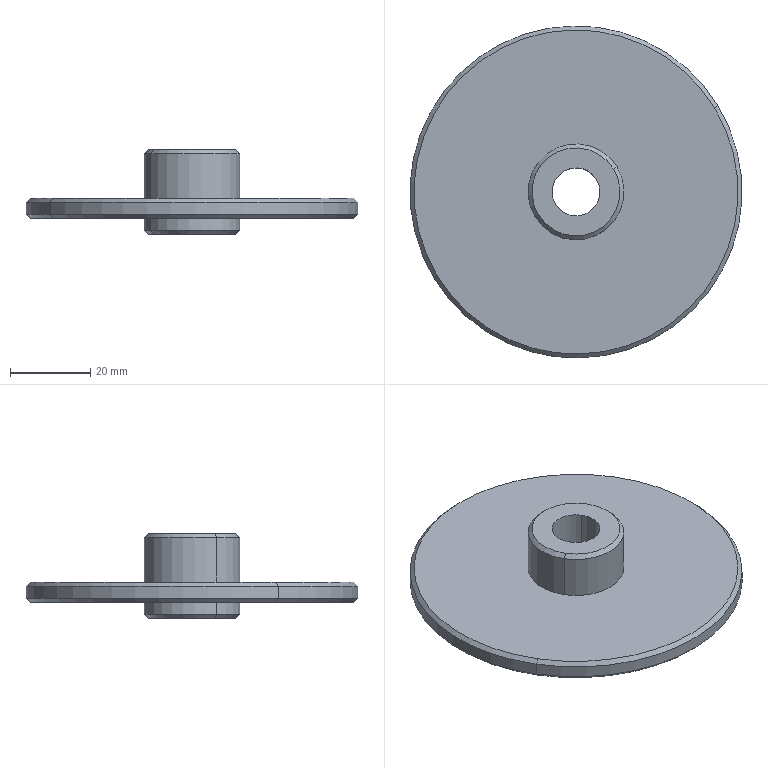Component | SolidWorks | TAR-02-033PaperStopWheel-1 | 1 solid | 20 faces | box 83 x 83 x 21 mm | volume 31584 mm3 | cone 8 | cylinder 8 | plane 4 | commonest cylinder face diameters 24 x4 12 x2 83 x2
build123d program:
from build123d import *

# Parameters (mm, degrees)
SKETCH1_R           = 12
BOSS_EXTRUDE1_DEPTH = 4
SKETCH2_R           = 41.5
BOSS_EXTRUDE2_DEPTH = 5
SKETCH3_R           = 12
BOSS_EXTRUDE3_DEPTH = 12
SKETCH4_R           = 6
CUT_EXTRUDE1_DEPTH  = 99
CHAMFER1_SIZE       = 1


with BuildPart() as part:
    # Sketch1 → Boss-Extrude1 (new body)
    with BuildSketch(Plane.XY):
        Circle(SKETCH1_R)
    extrude(amount=BOSS_EXTRUDE1_DEPTH)

    # Sketch2 → Boss-Extrude2 (add)
    with BuildSketch(Plane.XY.offset(4)):
        Circle(SKETCH2_R)
    extrude(amount=BOSS_EXTRUDE2_DEPTH)

    # Sketch3 → Boss-Extrude3 (add)
    with BuildSketch(Plane.XY.offset(9)):
        Circle(SKETCH3_R)
    extrude(amount=BOSS_EXTRUDE3_DEPTH)

    # Sketch4 → Cut-Extrude1 (cut)
    with BuildSketch(Plane.XY.offset(21)):
        Circle(SKETCH4_R)
    extrude(amount=-CUT_EXTRUDE1_DEPTH, mode=Mode.SUBTRACT)

    # Chamfer1
    chamfer1_edges = [part.edges().sort_by_distance(p)[0] for p in [
        (-12, 0, 21),
        (-12, 0, 0),
        (-41.5, 0, 4),
        (-41.5, 0, 9),
    ]]
    chamfer(chamfer1_edges, length=CHAMFER1_SIZE)


solid = part.part

# Placed as in the assembly
solid = solid.moved(Location((-115.391, 9.288, -85.4), (0, 0, 0)))
STEP:
#1=COLOUR_RGB('',0.7922,0.8196,0.9333);
#2=FILL_AREA_STYLE_COLOUR('',#1);
#3=FILL_AREA_STYLE('',(#2));
#4=SURFACE_STYLE_FILL_AREA(#3);
#5=SURFACE_SIDE_STYLE('',(#4));
#6=SURFACE_STYLE_USAGE(.BOTH.,#5);
#7=PRESENTATION_STYLE_ASSIGNMENT((#6));
#8=CARTESIAN_POINT('',(-4.173,0.5905,-2.535));
#9=VERTEX_POINT('',#8);
#10=CARTESIAN_POINT('',(-4.913,0.1408,-2.535));
#11=VERTEX_POINT('',#10);
#12=CARTESIAN_POINT('',(-4.543,0.3657,-2.535));
#13=DIRECTION('',(0.,0.,1.));
#14=DIRECTION('',(0.8546,0.5192,0.));
#15=AXIS2_PLACEMENT_3D('',#12,#13,#14);
#16=CIRCLE('',#15,0.4331);
#17=EDGE_CURVE('',#9,#11,#16,.T.);
#18=ORIENTED_EDGE('',*,*,#17,.F.);
#19=CARTESIAN_POINT('',(-4.139,0.611,-2.575));
#20=VERTEX_POINT('',#19);
#21=CARTESIAN_POINT('',(-4.173,0.5905,-2.535));
#22=DIRECTION('',(0.6043,0.3671,-0.7071));
#23=VECTOR('',#22,39.37);
#24=LINE('',#21,#23);
#25=EDGE_CURVE('',#9,#20,#24,.T.);
#26=ORIENTED_EDGE('',*,*,#25,.T.);
#27=CARTESIAN_POINT('',(-4.947,0.1204,-2.575));
#28=VERTEX_POINT('',#27);
#29=CARTESIAN_POINT('',(-4.543,0.3657,-2.575));
#30=DIRECTION('',(0.,0.,-1.));
#31=DIRECTION('',(0.8546,0.5192,0.));
#32=AXIS2_PLACEMENT_3D('',#29,#30,#31);
#33=CIRCLE('',#32,0.4724);
#34=EDGE_CURVE('',#28,#20,#33,.T.);
#35=ORIENTED_EDGE('',*,*,#34,.F.);
#36=CARTESIAN_POINT('',(-4.913,0.1408,-2.535));
#37=DIRECTION('',(-0.6043,-0.3671,-0.7071));
#38=VECTOR('',#37,39.37);
#39=LINE('',#36,#38);
#40=EDGE_CURVE('',#11,#28,#39,.T.);
#41=ORIENTED_EDGE('',*,*,#40,.F.);
#42=EDGE_LOOP('',(#18,#26,#35,#41));
#43=FACE_OUTER_BOUND('',#42,.T.);
#44=CARTESIAN_POINT('',(-4.543,0.3657,-2.535));
#45=DIRECTION('',(0.,0.,-1.));
#46=DIRECTION('',(-0.8546,-0.5192,0.));
#47=AXIS2_PLACEMENT_3D('',#44,#45,#46);
#48=CONICAL_SURFACE('',#47,0.4331,0.7854);
#49=ADVANCED_FACE('',(#43),#48,.T.);
#50=CARTESIAN_POINT('',(-4.913,0.1408,-3.362));
#51=VERTEX_POINT('',#50);
#52=CARTESIAN_POINT('',(-4.173,0.5905,-3.362));
#53=VERTEX_POINT('',#52);
#54=CARTESIAN_POINT('',(-4.543,0.3657,-3.362));
#55=DIRECTION('',(0.,0.,-1.));
#56=DIRECTION('',(0.8546,0.5192,0.));
#57=AXIS2_PLACEMENT_3D('',#54,#55,#56);
#58=CIRCLE('',#57,0.4331);
#59=EDGE_CURVE('',#51,#53,#58,.T.);
#60=ORIENTED_EDGE('',*,*,#59,.F.);
#61=CARTESIAN_POINT('',(-4.947,0.1204,-3.323));
#62=VERTEX_POINT('',#61);
#63=CARTESIAN_POINT('',(-4.947,0.1204,-3.323));
#64=DIRECTION('',(-0.6043,-0.3671,0.7071));
#65=VECTOR('',#64,39.37);
#66=LINE('',#63,#65);
#67=EDGE_CURVE('',#51,#62,#66,.T.);
#68=ORIENTED_EDGE('',*,*,#67,.T.);
#69=CARTESIAN_POINT('',(-4.139,0.611,-3.323));
#70=VERTEX_POINT('',#69);
#71=CARTESIAN_POINT('',(-4.543,0.3657,-3.323));
#72=DIRECTION('',(0.,0.,1.));
#73=DIRECTION('',(0.8546,0.5192,0.));
#74=AXIS2_PLACEMENT_3D('',#71,#72,#73);
#75=CIRCLE('',#74,0.4724);
#76=EDGE_CURVE('',#70,#62,#75,.T.);
#77=ORIENTED_EDGE('',*,*,#76,.F.);
#78=CARTESIAN_POINT('',(-4.139,0.611,-3.323));
#79=DIRECTION('',(0.6043,0.3671,0.7071));
#80=VECTOR('',#79,39.37);
#81=LINE('',#78,#80);
#82=EDGE_CURVE('',#53,#70,#81,.T.);
#83=ORIENTED_EDGE('',*,*,#82,.F.);
#84=EDGE_LOOP('',(#60,#68,#77,#83));
#85=FACE_OUTER_BOUND('',#84,.T.);
#86=CARTESIAN_POINT('',(-4.543,0.3657,-3.323));
#87=DIRECTION('',(0.,0.,1.));
#88=DIRECTION('',(0.8546,0.5192,0.));
#89=AXIS2_PLACEMENT_3D('',#86,#87,#88);
#90=CONICAL_SURFACE('',#89,0.4724,0.7854);
#91=ADVANCED_FACE('',(#85),#90,.T.);
#92=CARTESIAN_POINT('',(-3.18,1.194,-3.008));
#93=VERTEX_POINT('',#92);
#94=CARTESIAN_POINT('',(-5.906,-0.4622,-3.008));
#95=VERTEX_POINT('',#94);
#96=CARTESIAN_POINT('',(-4.543,0.3657,-3.008));
#97=DIRECTION('',(0.,0.,1.));
#98=DIRECTION('',(0.8546,0.5192,0.));
#99=AXIS2_PLACEMENT_3D('',#96,#97,#98);
#100=CIRCLE('',#99,1.594);
#101=EDGE_CURVE('',#93,#95,#100,.T.);
#102=ORIENTED_EDGE('',*,*,#101,.F.);
#103=CARTESIAN_POINT('',(-3.147,1.214,-3.047));
#104=VERTEX_POINT('',#103);
#105=CARTESIAN_POINT('',(-3.18,1.194,-3.008));
#106=DIRECTION('',(0.6043,0.3671,-0.7071));
#107=VECTOR('',#106,39.37);
#108=LINE('',#105,#107);
#109=EDGE_CURVE('',#93,#104,#108,.T.);
#110=ORIENTED_EDGE('',*,*,#109,.T.);
#111=CARTESIAN_POINT('',(-5.939,-0.4827,-3.047));
#112=VERTEX_POINT('',#111);
#113=CARTESIAN_POINT('',(-4.543,0.3657,-3.047));
#114=DIRECTION('',(0.,0.,-1.));
#115=DIRECTION('',(0.8546,0.5192,0.));
#116=AXIS2_PLACEMENT_3D('',#113,#114,#115);
#117=CIRCLE('',#116,1.634);
#118=EDGE_CURVE('',#112,#104,#117,.T.);
#119=ORIENTED_EDGE('',*,*,#118,.F.);
#120=CARTESIAN_POINT('',(-5.906,-0.4622,-3.008));
#121=DIRECTION('',(-0.6043,-0.3671,-0.7071));
#122=VECTOR('',#121,39.37);
#123=LINE('',#120,#122);
#124=EDGE_CURVE('',#95,#112,#123,.T.);
#125=ORIENTED_EDGE('',*,*,#124,.F.);
#126=EDGE_LOOP('',(#102,#110,#119,#125));
#127=FACE_OUTER_BOUND('',#126,.T.);
#128=CARTESIAN_POINT('',(-4.543,0.3657,-3.008));
#129=DIRECTION('',(0.,0.,-1.));
#130=DIRECTION('',(-0.8546,-0.5192,0.));
#131=AXIS2_PLACEMENT_3D('',#128,#129,#130);
#132=CONICAL_SURFACE('',#131,1.594,0.7854);
#133=ADVANCED_FACE('',(#127),#132,.T.);
#134=CARTESIAN_POINT('',(-5.906,-0.4622,-3.205));
#135=VERTEX_POINT('',#134);
#136=CARTESIAN_POINT('',(-3.18,1.194,-3.205));
#137=VERTEX_POINT('',#136);
#138=CARTESIAN_POINT('',(-4.543,0.3657,-3.205));
#139=DIRECTION('',(0.,0.,-1.));
#140=DIRECTION('',(0.8546,0.5192,0.));
#141=AXIS2_PLACEMENT_3D('',#138,#139,#140);
#142=CIRCLE('',#141,1.594);
#143=EDGE_CURVE('',#135,#137,#142,.T.);
#144=ORIENTED_EDGE('',*,*,#143,.F.);
#145=CARTESIAN_POINT('',(-5.939,-0.4827,-3.165));
#146=VERTEX_POINT('',#145);
#147=CARTESIAN_POINT('',(-5.939,-0.4827,-3.165));
#148=DIRECTION('',(-0.6043,-0.3671,0.7071));
#149=VECTOR('',#148,39.37);
#150=LINE('',#147,#149);
#151=EDGE_CURVE('',#135,#146,#150,.T.);
#152=ORIENTED_EDGE('',*,*,#151,.T.);
#153=CARTESIAN_POINT('',(-3.147,1.214,-3.165));
#154=VERTEX_POINT('',#153);
#155=CARTESIAN_POINT('',(-4.543,0.3657,-3.165));
#156=DIRECTION('',(0.,0.,1.));
#157=DIRECTION('',(0.8546,0.5192,0.));
#158=AXIS2_PLACEMENT_3D('',#155,#156,#157);
#159=CIRCLE('',#158,1.634);
#160=EDGE_CURVE('',#154,#146,#159,.T.);
#161=ORIENTED_EDGE('',*,*,#160,.F.);
#162=CARTESIAN_POINT('',(-3.147,1.214,-3.165));
#163=DIRECTION('',(0.6043,0.3671,0.7071));
#164=VECTOR('',#163,39.37);
#165=LINE('',#162,#164);
#166=EDGE_CURVE('',#137,#154,#165,.T.);
#167=ORIENTED_EDGE('',*,*,#166,.F.);
#168=EDGE_LOOP('',(#144,#152,#161,#167));
#169=FACE_OUTER_BOUND('',#168,.T.);
#170=CARTESIAN_POINT('',(-4.543,0.3657,-3.165));
#171=DIRECTION('',(0.,0.,1.));
#172=DIRECTION('',(0.8546,0.5192,0.));
#173=AXIS2_PLACEMENT_3D('',#170,#171,#172);
#174=CONICAL_SURFACE('',#173,1.634,0.7854);
#175=ADVANCED_FACE('',(#169),#174,.T.);
#176=CARTESIAN_POINT('',(-4.745,0.243,-3.362));
#177=VERTEX_POINT('',#176);
#178=CARTESIAN_POINT('',(-4.341,0.4883,-3.362));
#179=VERTEX_POINT('',#178);
#180=CARTESIAN_POINT('',(-4.543,0.3657,-3.362));
#181=DIRECTION('',(0.,0.,1.));
#182=DIRECTION('',(0.8546,0.5192,0.));
#183=AXIS2_PLACEMENT_3D('',#180,#181,#182);
#184=CIRCLE('',#183,0.2362);
#185=EDGE_CURVE('',#177,#179,#184,.T.);
#186=ORIENTED_EDGE('',*,*,#185,.F.);
#187=CARTESIAN_POINT('',(-4.745,0.243,-2.535));
#188=VERTEX_POINT('',#187);
#189=CARTESIAN_POINT('',(-4.745,0.243,-6.433));
#190=DIRECTION('',(0.,0.,1.));
#191=VECTOR('',#190,39.37);
#192=LINE('',#189,#191);
#193=EDGE_CURVE('',#177,#188,#192,.T.);
#194=ORIENTED_EDGE('',*,*,#193,.T.);
#195=CARTESIAN_POINT('',(-4.341,0.4883,-2.535));
#196=VERTEX_POINT('',#195);
#197=CARTESIAN_POINT('',(-4.543,0.3657,-2.535));
#198=DIRECTION('',(0.,0.,1.));
#199=DIRECTION('',(0.8546,0.5192,0.));
#200=AXIS2_PLACEMENT_3D('',#197,#198,#199);
#201=CIRCLE('',#200,0.2362);
#202=EDGE_CURVE('',#188,#196,#201,.T.);
#203=ORIENTED_EDGE('',*,*,#202,.T.);
#204=CARTESIAN_POINT('',(-4.341,0.4883,-6.433));
#205=DIRECTION('',(0.,0.,1.));
#206=VECTOR('',#205,39.37);
#207=LINE('',#204,#206);
#208=EDGE_CURVE('',#179,#196,#207,.T.);
#209=ORIENTED_EDGE('',*,*,#208,.F.);
#210=EDGE_LOOP('',(#186,#194,#203,#209));
#211=FACE_OUTER_BOUND('',#210,.T.);
#212=CARTESIAN_POINT('',(-4.543,0.3657,-6.433));
#213=DIRECTION('',(0.,0.,1.));
#214=DIRECTION('',(0.8546,0.5192,0.));
#215=AXIS2_PLACEMENT_3D('',#212,#213,#214);
#216=CYLINDRICAL_SURFACE('',#215,0.2362);
#217=ADVANCED_FACE('',(#211),#216,.F.);
#218=ORIENTED_EDGE('',*,*,#34,.T.);
#219=CARTESIAN_POINT('',(-4.139,0.611,-3.008));
#220=VERTEX_POINT('',#219);
#221=CARTESIAN_POINT('',(-4.139,0.611,-2.535));
#222=DIRECTION('',(0.,0.,-1.));
#223=VECTOR('',#222,39.37);
#224=LINE('',#221,#223);
#225=EDGE_CURVE('',#20,#220,#224,.T.);
#226=ORIENTED_EDGE('',*,*,#225,.T.);
#227=CARTESIAN_POINT('',(-4.947,0.1204,-3.008));
#228=VERTEX_POINT('',#227);
#229=CARTESIAN_POINT('',(-4.543,0.3657,-3.008));
#230=DIRECTION('',(0.,0.,1.));
#231=DIRECTION('',(0.8546,0.5192,0.));
#232=AXIS2_PLACEMENT_3D('',#229,#230,#231);
#233=CIRCLE('',#232,0.4724);
#234=EDGE_CURVE('',#220,#228,#233,.T.);
#235=ORIENTED_EDGE('',*,*,#234,.T.);
#236=CARTESIAN_POINT('',(-4.947,0.1204,-2.535));
#237=DIRECTION('',(0.,0.,-1.));
#238=VECTOR('',#237,39.37);
#239=LINE('',#236,#238);
#240=EDGE_CURVE('',#28,#228,#239,.T.);
#241=ORIENTED_EDGE('',*,*,#240,.F.);
#242=EDGE_LOOP('',(#218,#226,#235,#241));
#243=FACE_OUTER_BOUND('',#242,.T.);
#244=CARTESIAN_POINT('',(-4.543,0.3657,-2.535));
#245=DIRECTION('',(0.,0.,-1.));
#246=DIRECTION('',(-0.8546,-0.5192,0.));
#247=AXIS2_PLACEMENT_3D('',#244,#245,#246);
#248=CYLINDRICAL_SURFACE('',#247,0.4724);
#249=ADVANCED_FACE('',(#243),#248,.T.);
#250=ORIENTED_EDGE('',*,*,#118,.T.);
#251=CARTESIAN_POINT('',(-3.147,1.214,-3.008));
#252=DIRECTION('',(0.,0.,-1.));
#253=VECTOR('',#252,39.37);
#254=LINE('',#251,#253);
#255=EDGE_CURVE('',#104,#154,#254,.T.);
#256=ORIENTED_EDGE('',*,*,#255,.T.);
#257=ORIENTED_EDGE('',*,*,#160,.T.);
#258=CARTESIAN_POINT('',(-5.939,-0.4827,-3.008));
#259=DIRECTION('',(0.,0.,-1.));
#260=VECTOR('',#259,39.37);
#261=LINE('',#258,#260);
#262=EDGE_CURVE('',#112,#146,#261,.T.);
#263=ORIENTED_EDGE('',*,*,#262,.F.);
#264=EDGE_LOOP('',(#250,#256,#257,#263));
#265=FACE_OUTER_BOUND('',#264,.T.);
#266=CARTESIAN_POINT('',(-4.543,0.3657,-3.008));
#267=DIRECTION('',(0.,0.,-1.));
#268=DIRECTION('',(-0.8546,-0.5192,0.));
#269=AXIS2_PLACEMENT_3D('',#266,#267,#268);
#270=CYLINDRICAL_SURFACE('',#269,1.634);
#271=ADVANCED_FACE('',(#265),#270,.T.);
#272=CARTESIAN_POINT('',(-4.139,0.611,-3.205));
#273=VERTEX_POINT('',#272);
#274=CARTESIAN_POINT('',(-4.947,0.1204,-3.205));
#275=VERTEX_POINT('',#274);
#276=CARTESIAN_POINT('',(-4.543,0.3657,-3.205));
#277=DIRECTION('',(0.,0.,1.));
#278=DIRECTION('',(0.8546,0.5192,0.));
#279=AXIS2_PLACEMENT_3D('',#276,#277,#278);
#280=CIRCLE('',#279,0.4724);
#281=EDGE_CURVE('',#273,#275,#280,.T.);
#282=ORIENTED_EDGE('',*,*,#281,.F.);
#283=CARTESIAN_POINT('',(-4.139,0.611,-3.205));
#284=DIRECTION('',(0.,0.,-1.));
#285=VECTOR('',#284,39.37);
#286=LINE('',#283,#285);
#287=EDGE_CURVE('',#273,#70,#286,.T.);
#288=ORIENTED_EDGE('',*,*,#287,.T.);
#289=ORIENTED_EDGE('',*,*,#76,.T.);
#290=CARTESIAN_POINT('',(-4.947,0.1204,-3.205));
#291=DIRECTION('',(0.,0.,-1.));
#292=VECTOR('',#291,39.37);
#293=LINE('',#290,#292);
#294=EDGE_CURVE('',#275,#62,#293,.T.);
#295=ORIENTED_EDGE('',*,*,#294,.F.);
#296=EDGE_LOOP('',(#282,#288,#289,#295));
#297=FACE_OUTER_BOUND('',#296,.T.);
#298=CARTESIAN_POINT('',(-4.543,0.3657,-3.205));
#299=DIRECTION('',(0.,0.,-1.));
#300=DIRECTION('',(-0.8546,-0.5192,0.));
#301=AXIS2_PLACEMENT_3D('',#298,#299,#300);
#302=CYLINDRICAL_SURFACE('',#301,0.4724);
#303=ADVANCED_FACE('',(#297),#302,.T.);
#304=ORIENTED_EDGE('',*,*,#287,.F.);
#305=CARTESIAN_POINT('',(-4.543,0.3657,-3.205));
#306=DIRECTION('',(0.,0.,1.));
#307=DIRECTION('',(0.8546,0.5192,0.));
#308=AXIS2_PLACEMENT_3D('',#305,#306,#307);
#309=CIRCLE('',#308,0.4724);
#310=EDGE_CURVE('',#275,#273,#309,.T.);
#311=ORIENTED_EDGE('',*,*,#310,.F.);
#312=ORIENTED_EDGE('',*,*,#294,.T.);
#313=CARTESIAN_POINT('',(-4.543,0.3657,-3.323));
#314=DIRECTION('',(0.,0.,1.));
#315=DIRECTION('',(0.8546,0.5192,0.));
#316=AXIS2_PLACEMENT_3D('',#313,#314,#315);
#317=CIRCLE('',#316,0.4724);
#318=EDGE_CURVE('',#62,#70,#317,.T.);
#319=ORIENTED_EDGE('',*,*,#318,.T.);
#320=EDGE_LOOP('',(#304,#311,#312,#319));
#321=FACE_OUTER_BOUND('',#320,.T.);
#322=CARTESIAN_POINT('',(-4.543,0.3657,-3.205));
#323=DIRECTION('',(0.,0.,-1.));
#324=DIRECTION('',(-0.8546,-0.5192,0.));
#325=AXIS2_PLACEMENT_3D('',#322,#323,#324);
#326=CYLINDRICAL_SURFACE('',#325,0.4724);
#327=ADVANCED_FACE('',(#321),#326,.T.);
#328=CARTESIAN_POINT('',(-4.543,0.3657,-3.362));
#329=DIRECTION('',(0.,0.,-1.));
#330=DIRECTION('',(0.8546,0.5192,0.));
#331=AXIS2_PLACEMENT_3D('',#328,#329,#330);
#332=CIRCLE('',#331,0.4331);
#333=EDGE_CURVE('',#53,#51,#332,.T.);
#334=ORIENTED_EDGE('',*,*,#333,.T.);
#335=ORIENTED_EDGE('',*,*,#59,.T.);
#336=EDGE_LOOP('',(#334,#335));
#337=FACE_OUTER_BOUND('',#336,.T.);
#338=CARTESIAN_POINT('',(-4.543,0.3657,-3.362));
#339=DIRECTION('',(0.,0.,1.));
#340=DIRECTION('',(0.8546,0.5192,0.));
#341=AXIS2_PLACEMENT_3D('',#338,#339,#340);
#342=CIRCLE('',#341,0.2362);
#343=EDGE_CURVE('',#179,#177,#342,.T.);
#344=ORIENTED_EDGE('',*,*,#343,.T.);
#345=ORIENTED_EDGE('',*,*,#185,.T.);
#346=EDGE_LOOP('',(#344,#345));
#347=FACE_BOUND('',#346,.T.);
#348=CARTESIAN_POINT('',(-4.543,0.3657,-3.362));
#349=DIRECTION('',(0.,0.,1.));
#350=DIRECTION('',(0.8546,0.5192,0.));
#351=AXIS2_PLACEMENT_3D('',#348,#349,#350);
#352=PLANE('',#351);
#353=ADVANCED_FACE('',(#337,#347),#352,.F.);
#354=ORIENTED_EDGE('',*,*,#255,.F.);
#355=CARTESIAN_POINT('',(-4.543,0.3657,-3.047));
#356=DIRECTION('',(0.,0.,-1.));
#357=DIRECTION('',(0.8546,0.5192,0.));
#358=AXIS2_PLACEMENT_3D('',#355,#356,#357);
#359=CIRCLE('',#358,1.634);
#360=EDGE_CURVE('',#104,#112,#359,.T.);
#361=ORIENTED_EDGE('',*,*,#360,.T.);
#362=ORIENTED_EDGE('',*,*,#262,.T.);
#363=CARTESIAN_POINT('',(-4.543,0.3657,-3.165));
#364=DIRECTION('',(0.,0.,1.));
#365=DIRECTION('',(0.8546,0.5192,0.));
#366=AXIS2_PLACEMENT_3D('',#363,#364,#365);
#367=CIRCLE('',#366,1.634);
#368=EDGE_CURVE('',#146,#154,#367,.T.);
#369=ORIENTED_EDGE('',*,*,#368,.T.);
#370=EDGE_LOOP('',(#354,#361,#362,#369));
#371=FACE_OUTER_BOUND('',#370,.T.);
#372=CARTESIAN_POINT('',(-4.543,0.3657,-3.008));
#373=DIRECTION('',(0.,0.,-1.));
#374=DIRECTION('',(-0.8546,-0.5192,0.));
#375=AXIS2_PLACEMENT_3D('',#372,#373,#374);
#376=CYLINDRICAL_SURFACE('',#375,1.634);
#377=ADVANCED_FACE('',(#371),#376,.T.);
#378=CARTESIAN_POINT('',(-4.543,0.3657,-3.008));
#379=DIRECTION('',(0.,0.,1.));
#380=DIRECTION('',(0.8546,0.5192,0.));
#381=AXIS2_PLACEMENT_3D('',#378,#379,#380);
#382=CIRCLE('',#381,1.594);
#383=EDGE_CURVE('',#95,#93,#382,.T.);
#384=ORIENTED_EDGE('',*,*,#383,.T.);
#385=ORIENTED_EDGE('',*,*,#101,.T.);
#386=EDGE_LOOP('',(#384,#385));
#387=FACE_OUTER_BOUND('',#386,.T.);
#388=CARTESIAN_POINT('',(-4.543,0.3657,-3.008));
#389=DIRECTION('',(0.,0.,1.));
#390=DIRECTION('',(0.8546,0.5192,0.));
#391=AXIS2_PLACEMENT_3D('',#388,#389,#390);
#392=CIRCLE('',#391,0.4724);
#393=EDGE_CURVE('',#228,#220,#392,.T.);
#394=ORIENTED_EDGE('',*,*,#393,.F.);
#395=ORIENTED_EDGE('',*,*,#234,.F.);
#396=EDGE_LOOP('',(#394,#395));
#397=FACE_BOUND('',#396,.T.);
#398=CARTESIAN_POINT('',(-4.543,0.3657,-3.008));
#399=DIRECTION('',(0.,0.,1.));
#400=DIRECTION('',(0.8546,0.5192,0.));
#401=AXIS2_PLACEMENT_3D('',#398,#399,#400);
#402=PLANE('',#401);
#403=ADVANCED_FACE('',(#387,#397),#402,.T.);
#404=CARTESIAN_POINT('',(-4.543,0.3657,-3.205));
#405=DIRECTION('',(0.,0.,-1.));
#406=DIRECTION('',(0.8546,0.5192,0.));
#407=AXIS2_PLACEMENT_3D('',#404,#405,#406);
#408=CIRCLE('',#407,1.594);
#409=EDGE_CURVE('',#137,#135,#408,.T.);
#410=ORIENTED_EDGE('',*,*,#409,.T.);
#411=ORIENTED_EDGE('',*,*,#143,.T.);
#412=EDGE_LOOP('',(#410,#411));
#413=FACE_OUTER_BOUND('',#412,.T.);
#414=ORIENTED_EDGE('',*,*,#310,.T.);
#415=ORIENTED_EDGE('',*,*,#281,.T.);
#416=EDGE_LOOP('',(#414,#415));
#417=FACE_BOUND('',#416,.T.);
#418=CARTESIAN_POINT('',(-4.543,0.3657,-3.205));
#419=DIRECTION('',(0.,0.,1.));
#420=DIRECTION('',(0.8546,0.5192,0.));
#421=AXIS2_PLACEMENT_3D('',#418,#419,#420);
#422=PLANE('',#421);
#423=ADVANCED_FACE('',(#413,#417),#422,.F.);
#424=ORIENTED_EDGE('',*,*,#225,.F.);
#425=CARTESIAN_POINT('',(-4.543,0.3657,-2.575));
#426=DIRECTION('',(0.,0.,-1.));
#427=DIRECTION('',(0.8546,0.5192,0.));
#428=AXIS2_PLACEMENT_3D('',#425,#426,#427);
#429=CIRCLE('',#428,0.4724);
#430=EDGE_CURVE('',#20,#28,#429,.T.);
#431=ORIENTED_EDGE('',*,*,#430,.T.);
#432=ORIENTED_EDGE('',*,*,#240,.T.);
#433=ORIENTED_EDGE('',*,*,#393,.T.);
#434=EDGE_LOOP('',(#424,#431,#432,#433));
#435=FACE_OUTER_BOUND('',#434,.T.);
#436=CARTESIAN_POINT('',(-4.543,0.3657,-2.535));
#437=DIRECTION('',(0.,0.,-1.));
#438=DIRECTION('',(-0.8546,-0.5192,0.));
#439=AXIS2_PLACEMENT_3D('',#436,#437,#438);
#440=CYLINDRICAL_SURFACE('',#439,0.4724);
#441=ADVANCED_FACE('',(#435),#440,.T.);
#442=CARTESIAN_POINT('',(-4.543,0.3657,-2.535));
#443=DIRECTION('',(0.,0.,1.));
#444=DIRECTION('',(0.8546,0.5192,0.));
#445=AXIS2_PLACEMENT_3D('',#442,#443,#444);
#446=CIRCLE('',#445,0.4331);
#447=EDGE_CURVE('',#11,#9,#446,.T.);
#448=ORIENTED_EDGE('',*,*,#447,.T.);
#449=ORIENTED_EDGE('',*,*,#17,.T.);
#450=EDGE_LOOP('',(#448,#449));
#451=FACE_OUTER_BOUND('',#450,.T.);
#452=CARTESIAN_POINT('',(-4.543,0.3657,-2.535));
#453=DIRECTION('',(0.,0.,1.));
#454=DIRECTION('',(0.8546,0.5192,0.));
#455=AXIS2_PLACEMENT_3D('',#452,#453,#454);
#456=CIRCLE('',#455,0.2362);
#457=EDGE_CURVE('',#196,#188,#456,.T.);
#458=ORIENTED_EDGE('',*,*,#457,.F.);
#459=ORIENTED_EDGE('',*,*,#202,.F.);
#460=EDGE_LOOP('',(#458,#459));
#461=FACE_BOUND('',#460,.T.);
#462=CARTESIAN_POINT('',(-4.543,0.3657,-2.535));
#463=DIRECTION('',(0.,0.,1.));
#464=DIRECTION('',(0.8546,0.5192,0.));
#465=AXIS2_PLACEMENT_3D('',#462,#463,#464);
#466=PLANE('',#465);
#467=ADVANCED_FACE('',(#451,#461),#466,.T.);
#468=ORIENTED_EDGE('',*,*,#193,.F.);
#469=ORIENTED_EDGE('',*,*,#343,.F.);
#470=ORIENTED_EDGE('',*,*,#208,.T.);
#471=ORIENTED_EDGE('',*,*,#457,.T.);
#472=EDGE_LOOP('',(#468,#469,#470,#471));
#473=FACE_OUTER_BOUND('',#472,.T.);
#474=CARTESIAN_POINT('',(-4.543,0.3657,-6.433));
#475=DIRECTION('',(0.,0.,1.));
#476=DIRECTION('',(0.8546,0.5192,0.));
#477=AXIS2_PLACEMENT_3D('',#474,#475,#476);
#478=CYLINDRICAL_SURFACE('',#477,0.2362);
#479=ADVANCED_FACE('',(#473),#478,.F.);
#480=ORIENTED_EDGE('',*,*,#151,.F.);
#481=ORIENTED_EDGE('',*,*,#409,.F.);
#482=ORIENTED_EDGE('',*,*,#166,.T.);
#483=ORIENTED_EDGE('',*,*,#368,.F.);
#484=EDGE_LOOP('',(#480,#481,#482,#483));
#485=FACE_OUTER_BOUND('',#484,.T.);
#486=CARTESIAN_POINT('',(-4.543,0.3657,-3.165));
#487=DIRECTION('',(0.,0.,1.));
#488=DIRECTION('',(0.8546,0.5192,0.));
#489=AXIS2_PLACEMENT_3D('',#486,#487,#488);
#490=CONICAL_SURFACE('',#489,1.634,0.7854);
#491=ADVANCED_FACE('',(#485),#490,.T.);
#492=ORIENTED_EDGE('',*,*,#109,.F.);
#493=ORIENTED_EDGE('',*,*,#383,.F.);
#494=ORIENTED_EDGE('',*,*,#124,.T.);
#495=ORIENTED_EDGE('',*,*,#360,.F.);
#496=EDGE_LOOP('',(#492,#493,#494,#495));
#497=FACE_OUTER_BOUND('',#496,.T.);
#498=CARTESIAN_POINT('',(-4.543,0.3657,-3.008));
#499=DIRECTION('',(0.,0.,-1.));
#500=DIRECTION('',(-0.8546,-0.5192,0.));
#501=AXIS2_PLACEMENT_3D('',#498,#499,#500);
#502=CONICAL_SURFACE('',#501,1.594,0.7854);
#503=ADVANCED_FACE('',(#497),#502,.T.);
#504=ORIENTED_EDGE('',*,*,#67,.F.);
#505=ORIENTED_EDGE('',*,*,#333,.F.);
#506=ORIENTED_EDGE('',*,*,#82,.T.);
#507=ORIENTED_EDGE('',*,*,#318,.F.);
#508=EDGE_LOOP('',(#504,#505,#506,#507));
#509=FACE_OUTER_BOUND('',#508,.T.);
#510=CARTESIAN_POINT('',(-4.543,0.3657,-3.323));
#511=DIRECTION('',(0.,0.,1.));
#512=DIRECTION('',(0.8546,0.5192,0.));
#513=AXIS2_PLACEMENT_3D('',#510,#511,#512);
#514=CONICAL_SURFACE('',#513,0.4724,0.7854);
#515=ADVANCED_FACE('',(#509),#514,.T.);
#516=ORIENTED_EDGE('',*,*,#25,.F.);
#517=ORIENTED_EDGE('',*,*,#447,.F.);
#518=ORIENTED_EDGE('',*,*,#40,.T.);
#519=ORIENTED_EDGE('',*,*,#430,.F.);
#520=EDGE_LOOP('',(#516,#517,#518,#519));
#521=FACE_OUTER_BOUND('',#520,.T.);
#522=CARTESIAN_POINT('',(-4.543,0.3657,-2.535));
#523=DIRECTION('',(0.,0.,-1.));
#524=DIRECTION('',(-0.8546,-0.5192,0.));
#525=AXIS2_PLACEMENT_3D('',#522,#523,#524);
#526=CONICAL_SURFACE('',#525,0.4331,0.7854);
#527=ADVANCED_FACE('',(#521),#526,.T.);
#528=CLOSED_SHELL('',(#49,#91,#133,#175,#217,#249,#271,#303,#327,#353,#377,#403,#423,#441,#467,#479,#491,#503,#515,#527));
#529=MANIFOLD_SOLID_BREP('',#528);
#530=STYLED_ITEM('',(#7),#529);
#531=(LENGTH_UNIT()NAMED_UNIT(*)SI_UNIT($,.METRE.));
#532=LENGTH_MEASURE_WITH_UNIT(LENGTH_MEASURE(0.0254),#531);
#533=DIMENSIONAL_EXPONENTS(1.,0.,0.,0.,0.,0.,0.);
#534=(CONVERSION_BASED_UNIT('',#532)LENGTH_UNIT()NAMED_UNIT(#533));
#535=UNCERTAINTY_MEASURE_WITH_UNIT(LENGTH_MEASURE(0.00001),#534,'','');
#536=(NAMED_UNIT(*)PLANE_ANGLE_UNIT()SI_UNIT($,.RADIAN.));
#537=(NAMED_UNIT(*)SI_UNIT($,.STERADIAN.)SOLID_ANGLE_UNIT());
#538=(GEOMETRIC_REPRESENTATION_CONTEXT(3)GLOBAL_UNCERTAINTY_ASSIGNED_CONTEXT((#535))GLOBAL_UNIT_ASSIGNED_CONTEXT((#534,#536,#537))REPRESENTATION_CONTEXT('',''));
#539=MECHANICAL_DESIGN_GEOMETRIC_PRESENTATION_REPRESENTATION('',(#530),#538);
#540=PRESENTATION_LAYER_ASSIGNMENT('','',(#530));
#541=CARTESIAN_POINT('',(0.,0.,0.));
#542=DIRECTION('',(0.,0.,1.));
#543=DIRECTION('',(1.,0.,0.));
#544=AXIS2_PLACEMENT_3D('',#541,#542,#543);
#545=(LENGTH_UNIT()NAMED_UNIT(*)SI_UNIT($,.METRE.));
#546=LENGTH_MEASURE_WITH_UNIT(LENGTH_MEASURE(0.0254),#545);
#547=DIMENSIONAL_EXPONENTS(1.,0.,0.,0.,0.,0.,0.);
#548=(CONVERSION_BASED_UNIT('',#546)LENGTH_UNIT()NAMED_UNIT(#547));
#549=UNCERTAINTY_MEASURE_WITH_UNIT(LENGTH_MEASURE(0.00001),#548,'','');
#550=(NAMED_UNIT(*)PLANE_ANGLE_UNIT()SI_UNIT($,.RADIAN.));
#551=(NAMED_UNIT(*)SI_UNIT($,.STERADIAN.)SOLID_ANGLE_UNIT());
#552=(GEOMETRIC_REPRESENTATION_CONTEXT(3)GLOBAL_UNCERTAINTY_ASSIGNED_CONTEXT((#549))GLOBAL_UNIT_ASSIGNED_CONTEXT((#548,#550,#551))REPRESENTATION_CONTEXT('',''));
#553=ADVANCED_BREP_SHAPE_REPRESENTATION('',(#529,#544),#552);